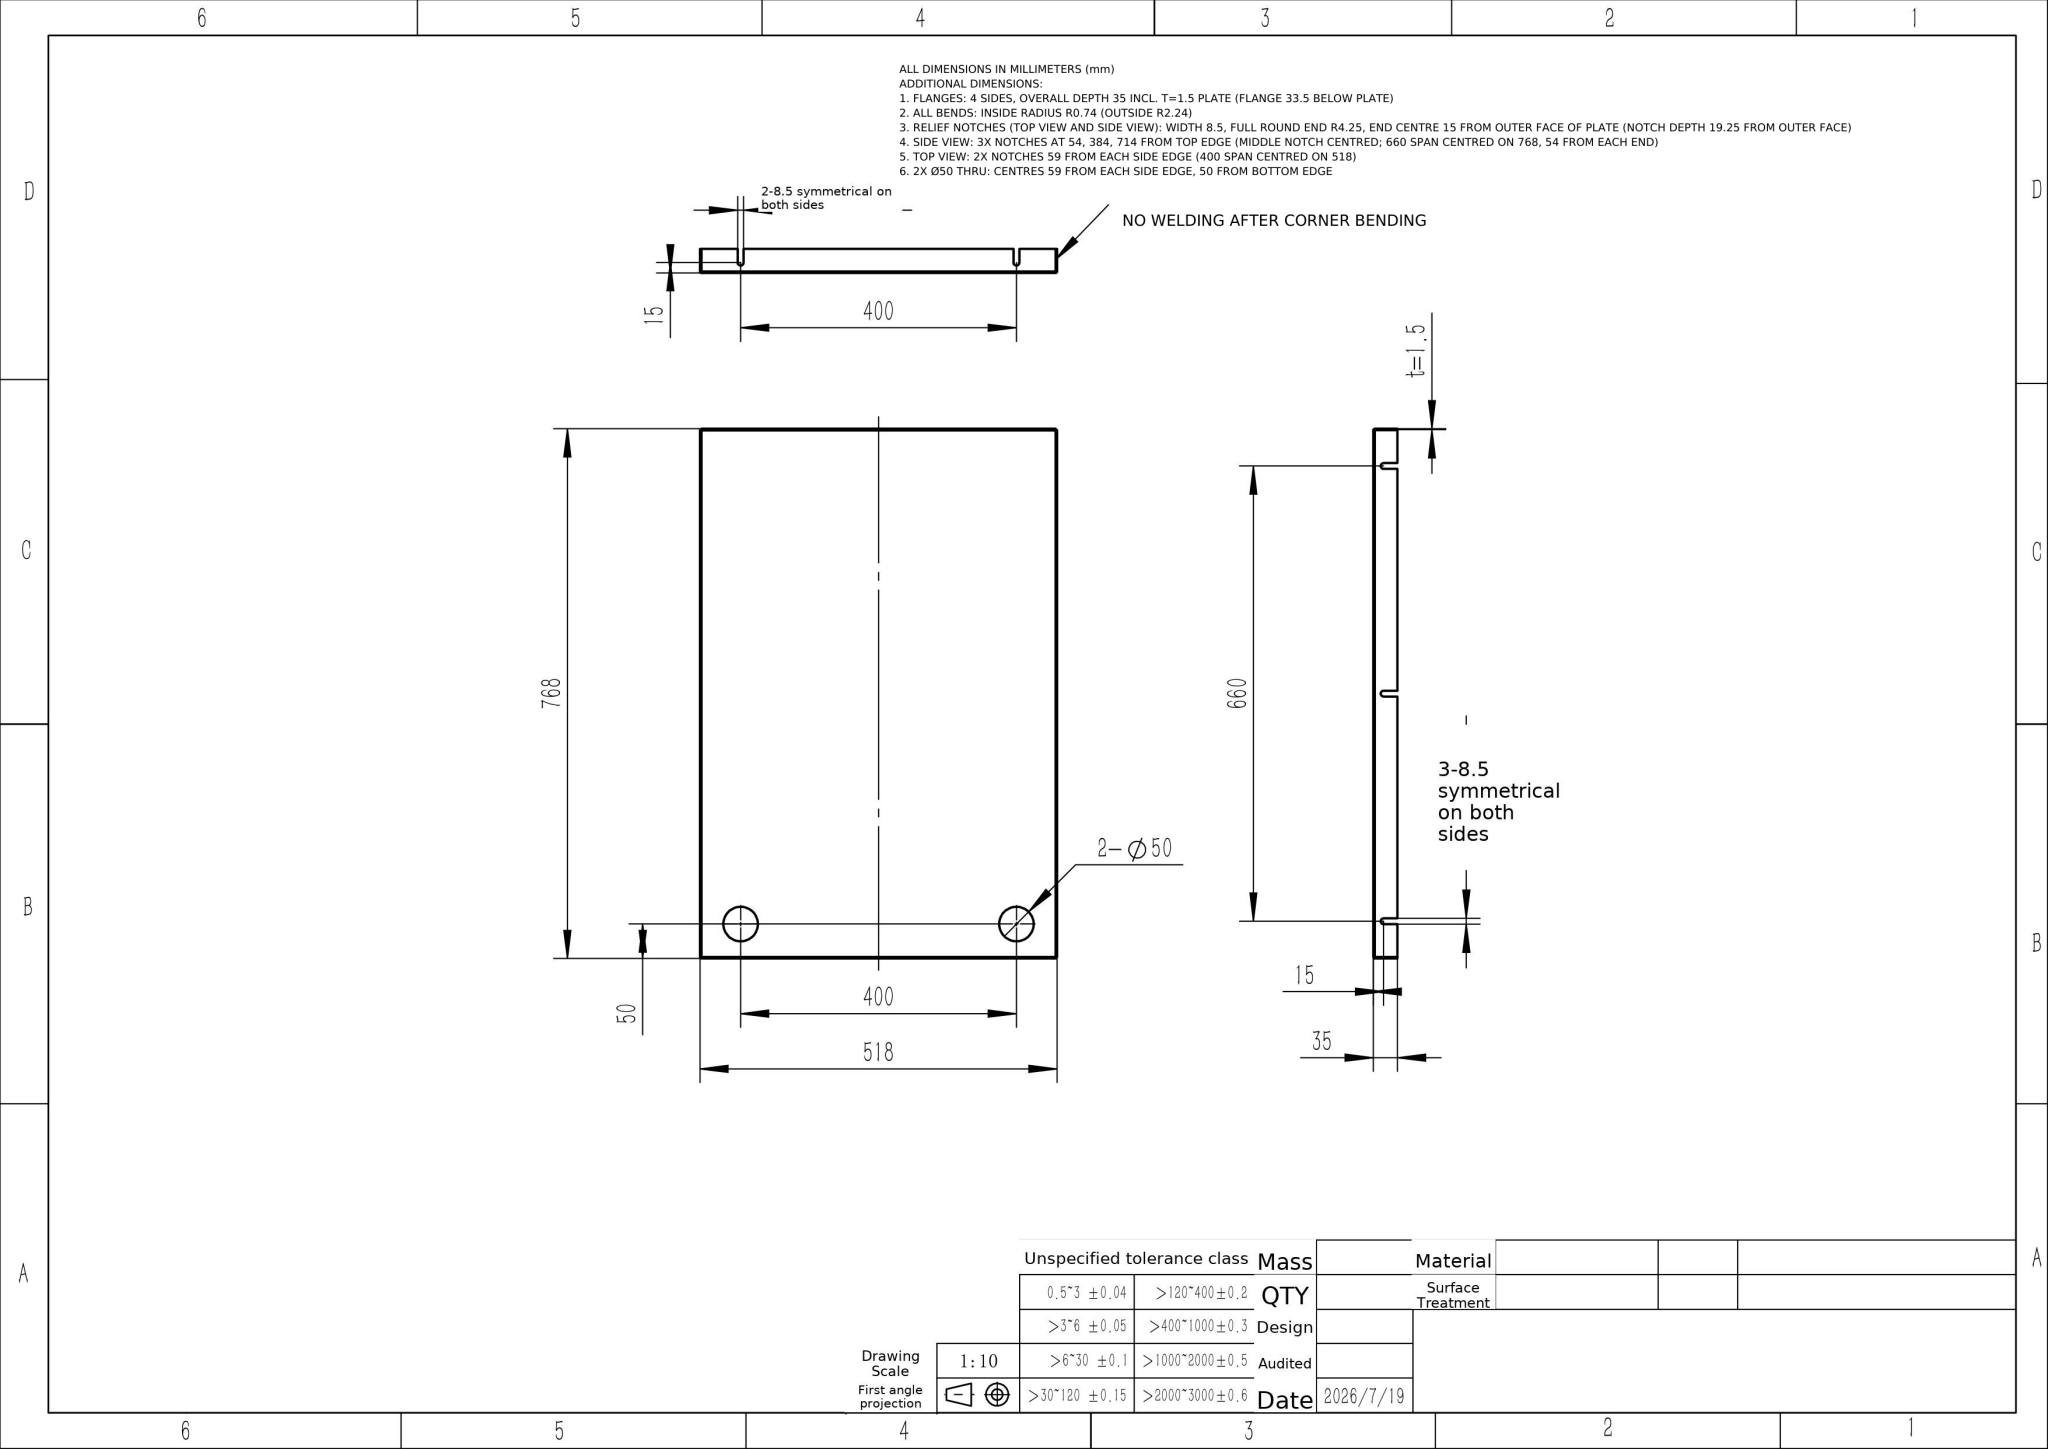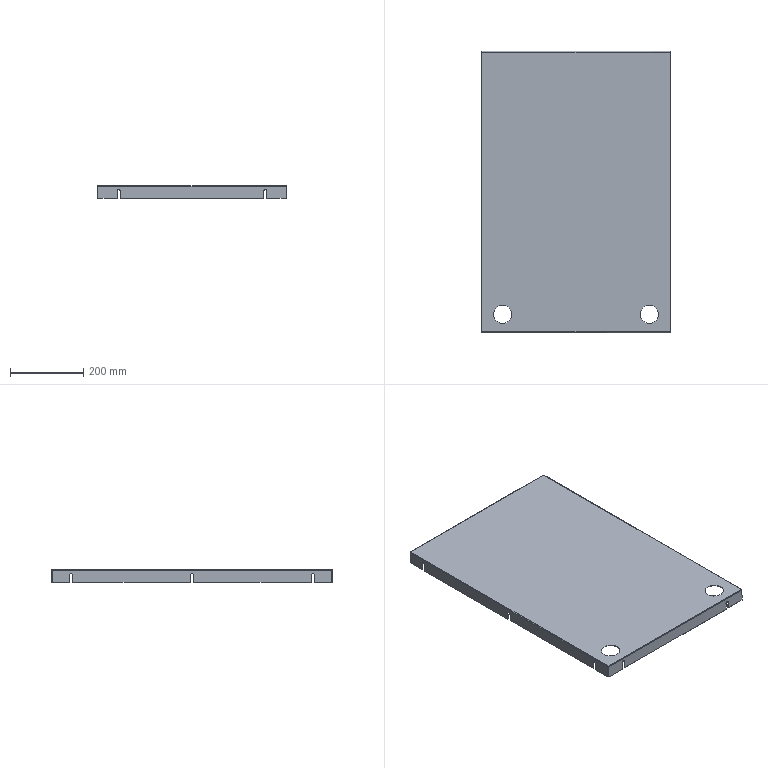Part | NX | mm | 1 solid | 86 faces | box 518 x 768 x 35 mm | volume 713751 mm3 | plane 52 | cylinder 26 | spline 8 | commonest cylinder face diameters 8.5 x14 50 x4 4.473 x4 1.473 x4